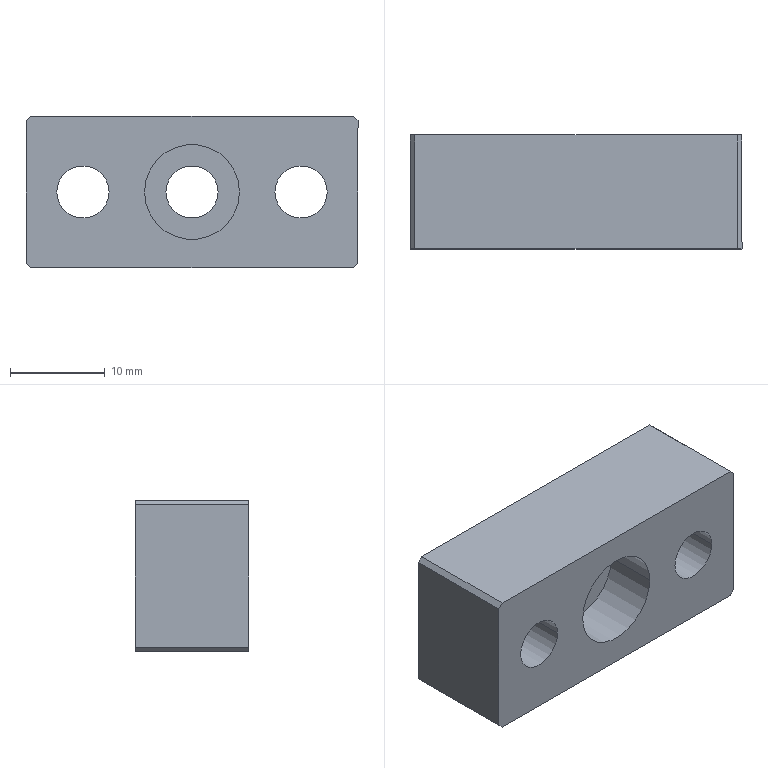Component | SolidWorks | 011-1 | 1 solid | 28 faces | box 35 x 12 x 16 mm | volume 4812 mm3 | cylinder 14 | plane 14 | commonest cylinder face diameters 10 x8 5.5 x6 | material AL6061
build123d program:
from build123d import *

# Parameters (mm, degrees)
SKETCH1_W                                         = 35
SKETCH1_H                                         = 16
BOSS_EXTRUDE1_DEPTH                               = 12
SKETCH2_R                                         = 5
CUT_EXTRUDE1_DEPTH                                = 2
HOLE_SIZE_ACCORDING_TO_TYPE_OF_HEX_SO_D           = 5.5
HOLE_SIZE_ACCORDING_TO_TYPE_OF_HEX_SO_DEPTH       = 22.18
HOLE_SIZE_ACCORDING_TO_TYPE_OF_HEX_SO_CBORE_D     = 10
HOLE_SIZE_ACCORDING_TO_TYPE_OF_HEX_SO_CBORE_DEPTH = 5.7
HOLE_SIZE_ACCORDING_TO_TYPE_OF_HEX_SO_TIP         = 1.652
HOLE_SIZE_ACCORDING_TO_TYPE_OF_HE_2_D             = 5.5
HOLE_SIZE_ACCORDING_TO_TYPE_OF_HE_2_DEPTH         = 22.18
HOLE_SIZE_ACCORDING_TO_TYPE_OF_HE_2_CBORE_D       = 10
HOLE_SIZE_ACCORDING_TO_TYPE_OF_HE_2_CBORE_DEPTH   = 5.7
HOLE_SIZE_ACCORDING_TO_TYPE_OF_HE_2_TIP           = 1.652
CHAMFER1_SIZE                                     = 0.5


with BuildPart() as part:
    # Sketch1 → Boss-Extrude1 (new body)
    with BuildSketch(Plane.XY):
        Rectangle(SKETCH1_W, SKETCH1_H)
    extrude(amount=BOSS_EXTRUDE1_DEPTH)

    # Sketch2 → Cut-Extrude1 (cut)
    with BuildSketch(Plane.XY.offset(12)):
        Circle(SKETCH2_R)
    extrude(amount=-CUT_EXTRUDE1_DEPTH, mode=Mode.SUBTRACT)

    # Hole Size _ according to_ type of hex so
    with Locations(Plane(origin=(0, 0, 0), x_dir=(-1, 0, 0), z_dir=(0, 0, -1))):
        with Locations((0, 0)):
            CounterBoreHole(HOLE_SIZE_ACCORDING_TO_TYPE_OF_HEX_SO_D / 2, HOLE_SIZE_ACCORDING_TO_TYPE_OF_HEX_SO_CBORE_D / 2, HOLE_SIZE_ACCORDING_TO_TYPE_OF_HEX_SO_CBORE_DEPTH, depth=HOLE_SIZE_ACCORDING_TO_TYPE_OF_HEX_SO_DEPTH)
            with Locations((0, 0, -(HOLE_SIZE_ACCORDING_TO_TYPE_OF_HEX_SO_DEPTH + HOLE_SIZE_ACCORDING_TO_TYPE_OF_HEX_SO_TIP / 2))):  # 118° drill point
                Cone(0, HOLE_SIZE_ACCORDING_TO_TYPE_OF_HEX_SO_D / 2, HOLE_SIZE_ACCORDING_TO_TYPE_OF_HEX_SO_TIP, mode=Mode.SUBTRACT)

    # Hole Size _ according to_ type of he 2
    with Locations(Plane.XY.offset(12)):
        with Locations((-11.5, 0), (11.5, 0)):
            CounterBoreHole(HOLE_SIZE_ACCORDING_TO_TYPE_OF_HE_2_D / 2, HOLE_SIZE_ACCORDING_TO_TYPE_OF_HE_2_CBORE_D / 2, HOLE_SIZE_ACCORDING_TO_TYPE_OF_HE_2_CBORE_DEPTH, depth=HOLE_SIZE_ACCORDING_TO_TYPE_OF_HE_2_DEPTH)
            with Locations((0, 0, -(HOLE_SIZE_ACCORDING_TO_TYPE_OF_HE_2_DEPTH + HOLE_SIZE_ACCORDING_TO_TYPE_OF_HE_2_TIP / 2))):  # 118° drill point
                Cone(0, HOLE_SIZE_ACCORDING_TO_TYPE_OF_HE_2_D / 2, HOLE_SIZE_ACCORDING_TO_TYPE_OF_HE_2_TIP, mode=Mode.SUBTRACT)

    # Chamfer1
    chamfer1_edges = [part.edges().sort_by_distance(p)[0] for p in [
        (17.5, -8, 6),
        (-17.5, -8, 6),
        (-17.5, 8, 6),
        (17.5, 8, 6),
    ]]
    chamfer(chamfer1_edges, length=CHAMFER1_SIZE)


solid = part.part

# Placed as in the assembly
solid = solid.moved(Location((-240.455, -163.942, -183.376), (-90, 0, 0)))